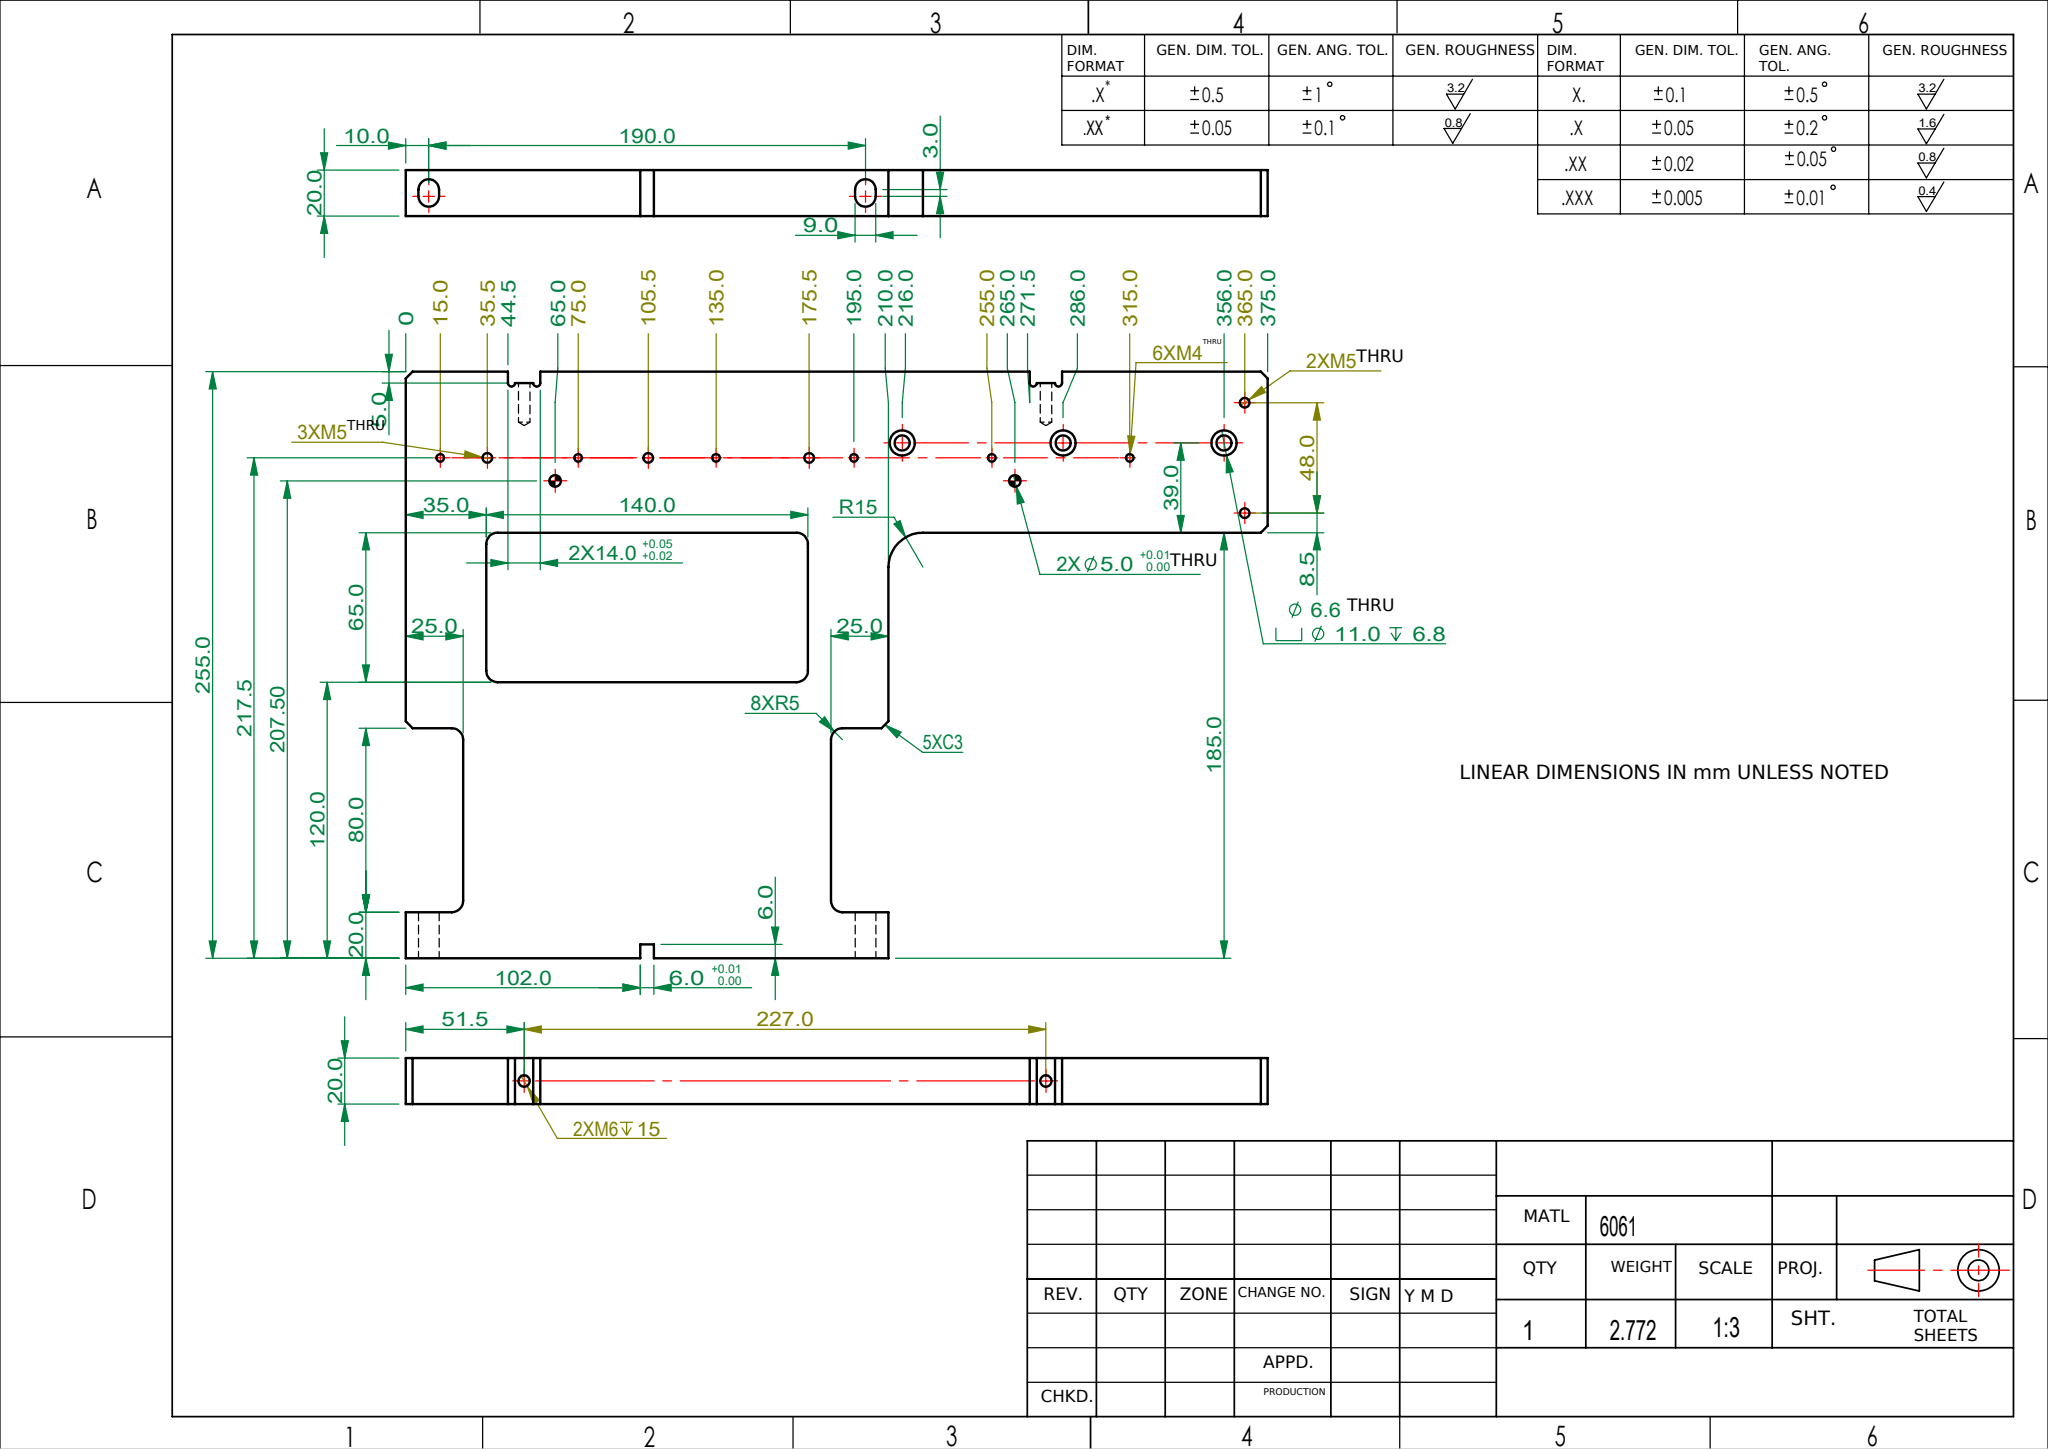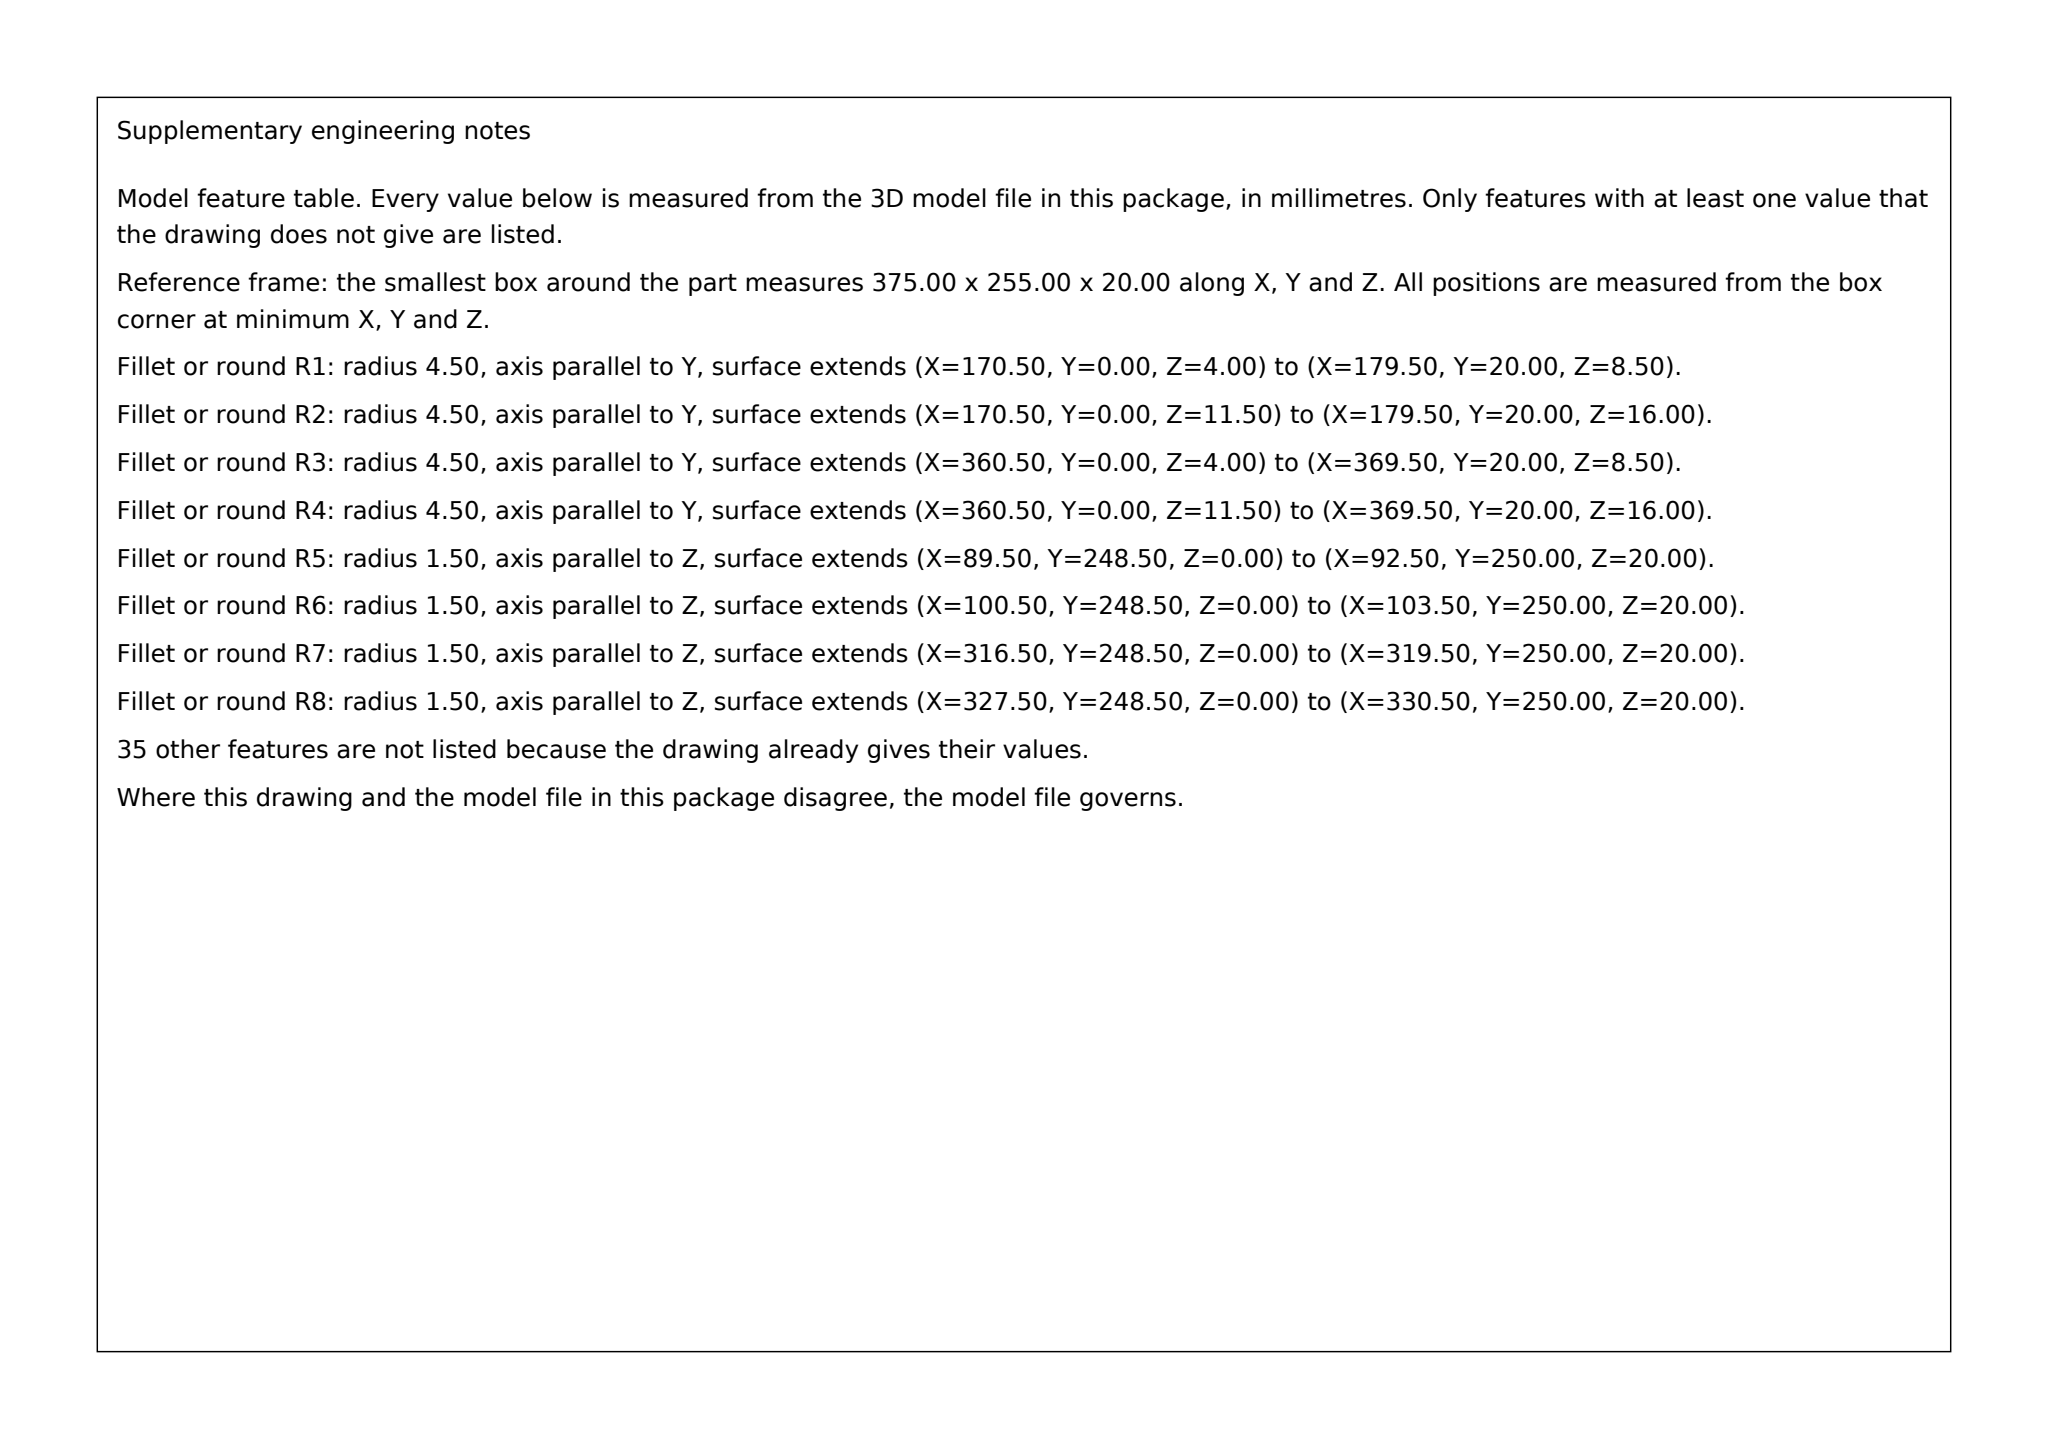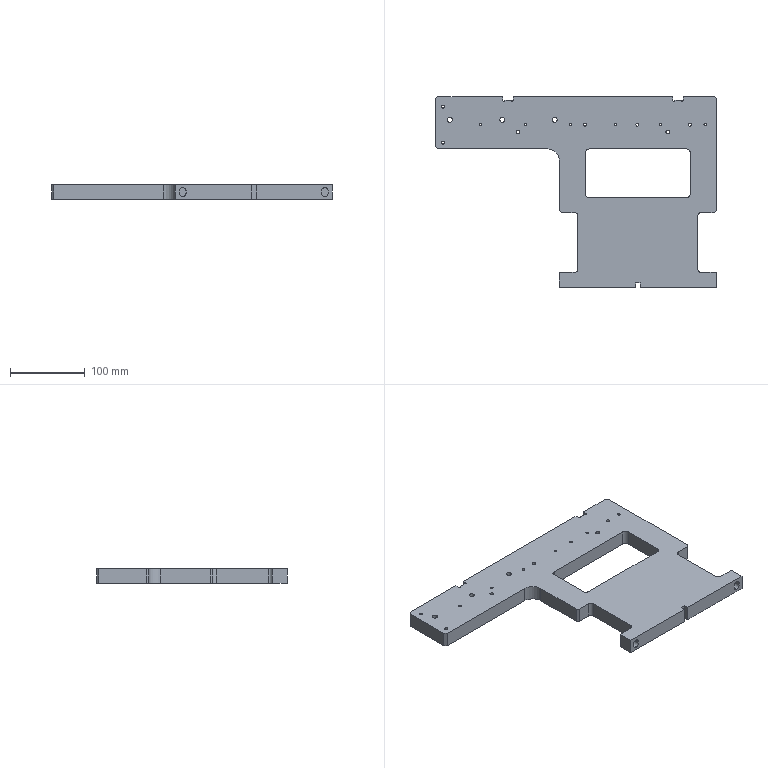Part | SolidWorks | mm | material 6061 | 1 solid | 109 faces | box 375 x 255 x 20 mm | volume 1026769 mm3 | cylinder 61 | plane 44 | cone 4 | commonest cylinder face diameters 3.3 x12 4.2 x10 5 x8 10 x8 11 x6 6.6 x6 9 x6 3 x4
build123d program:
from build123d import *

# Parameters (mm, degrees)
SKETCH1_W                                          = 375
SKETCH1_H                                          = 255
BOSS_EXTRUDE1_DEPTH                                = 20
M5_TAPPED_HOLE1_D                                  = 4.2
M4_TAPPED_HOLE1_D                                  = 3.3
LPATTERN1_COUNT                                    = 6
LPATTERN1_PITCH                                    = 60
SKETCH6_W                                          = 165
SKETCH6_H                                          = 185
CUT_EXTRUDE1_DEPTH                                 = 70
SKETCH7_W                                          = 25
SKETCH7_H                                          = 80
CUT_EXTRUDE2_DEPTH                                 = 70
F_8_5_8_5_DIAMETER_HOLE1_REACH                     = 447.365
F_8_5_8_5_DIAMETER_HOLE1_BORE_R                    = 4.25
CUT_EXTRUDE3_DEPTH                                 = 70
HOLE_SIZE_ACCORDING_TO_TYPE_1_OF_HEXAG_D           = 6.6
HOLE_SIZE_ACCORDING_TO_TYPE_1_OF_HEXAG_CBORE_D     = 11
HOLE_SIZE_ACCORDING_TO_TYPE_1_OF_HEXAG_CBORE_DEPTH = 6.8
LPATTERN2_COUNT                                    = 3
LPATTERN2_PITCH                                    = 70
SKETCH14_W                                         = 140
SKETCH14_H                                         = 65
CUT_EXTRUDE4_DEPTH                                 = 79
FILLET1_R                                          = 5
SKETCH17_W                                         = 14
SKETCH17_H                                         = 10
CUT_EXTRUDE5_DEPTH                                 = 37
LPATTERN3_COUNT                                    = 2
LPATTERN3_PITCH                                    = 227
SKETCH20_W                                         = 6
SKETCH20_H                                         = 12
CUT_EXTRUDE6_DEPTH                                 = 37
SIZE_MM_DOWEL_PIN_HOLE_1_D                         = 5
FILLET2_R                                          = 15
CHAMFER1_SIZE                                      = 3
FILLET3_R                                          = 5
M5_TAPPED_HOLE2_D                                  = 4.2
LPATTERN4_COUNT                                    = 3
LPATTERN4_PITCH                                    = 70
SKETCH25_R                                         = 1.5
CUT_EXTRUDE7_DEPTH                                 = 36


with BuildPart() as part:
    # Sketch1 → Boss-Extrude1 (new body)
    with BuildSketch(Plane.XY):
        Rectangle(SKETCH1_W, SKETCH1_H)
    extrude(amount=BOSS_EXTRUDE1_DEPTH)

    # M5 Tapped Hole1 (through all)
    with Locations(Plane(origin=(-177.5, 114, 20), x_dir=(1, 0, 0), z_dir=(0, 0, 1))):
        with Locations((0, 0), (0, -48)):
            Hole(M5_TAPPED_HOLE1_D / 2)

    # M4 Tapped Hole1 (through all)
    with Locations(Plane(origin=(-127.5, 90, 20), x_dir=(1, 0, 0), z_dir=(0, 0, 1))):
        with Locations((0, 0)):
            m4_tapped_hole1 = Hole(M4_TAPPED_HOLE1_D / 2)

    # LPattern1: M4 Tapped Hole1 ×6
    with Locations(*[(i * LPATTERN1_PITCH, 0, 0) for i in range(1, LPATTERN1_COUNT)]):
        add(m4_tapped_hole1, mode=Mode.SUBTRACT)

    # Sketch6 → Cut-Extrude1 (cut)
    with BuildSketch(Plane.XY.offset(20)):
        with Locations((-105, -35)):
            Rectangle(SKETCH6_W, SKETCH6_H)
    extrude(amount=-CUT_EXTRUDE1_DEPTH, mode=Mode.SUBTRACT)

    # Sketch7 → Cut-Extrude2 (cut)
    with BuildSketch(Plane.XY.offset(20)):
        with Locations((-10, -67.5)):
            Rectangle(SKETCH7_W, SKETCH7_H)
        with Locations((175, -67.5)):
            Rectangle(SKETCH7_W, SKETCH7_H)
    extrude(amount=-CUT_EXTRUDE2_DEPTH, mode=Mode.SUBTRACT)

    # 8.5 _8.5_ Diameter Hole1 bore (on position points) → 8.5 _8.5_ Diameter Hole1 (cut, up to next)
    with BuildSketch(Plane(origin=(177.5, -127.5, 10), x_dir=(0, 0, -1), z_dir=(0, -1, 0)), mode=Mode.PRIVATE) as f_8_5_8_5_diameter_hole1_sk1:
        Circle(F_8_5_8_5_DIAMETER_HOLE1_BORE_R)
    f_8_5_8_5_diameter_hole1_tool1 = extrude(f_8_5_8_5_diameter_hole1_sk1.sketch, amount=-F_8_5_8_5_DIAMETER_HOLE1_REACH, mode=Mode.PRIVATE) & part.part
    # 8.5 _8.5_ Diameter Hole1 bore (on position points) → 8.5 _8.5_ Diameter Hole1 (cut, up to next)
    with BuildSketch(Plane(origin=(177.5, -127.5, 10), x_dir=(0, 0, -1), z_dir=(0, -1, 0)), mode=Mode.PRIVATE) as f_8_5_8_5_diameter_hole1_sk2:
        with Locations((0, -190)):
            Circle(F_8_5_8_5_DIAMETER_HOLE1_BORE_R)
    f_8_5_8_5_diameter_hole1_tool2 = extrude(f_8_5_8_5_diameter_hole1_sk2.sketch, amount=-F_8_5_8_5_DIAMETER_HOLE1_REACH, mode=Mode.PRIVATE) & part.part
    add(f_8_5_8_5_diameter_hole1_tool1.solids().sort_by_distance((177.5, -127.5, 10))[0], mode=Mode.SUBTRACT)
    add(f_8_5_8_5_diameter_hole1_tool2.solids().sort_by_distance((-12.5, -127.5, 10))[0], mode=Mode.SUBTRACT)

    # Sketch11 → Cut-Extrude3 (cut)
    with BuildSketch(Plane.XZ.offset(127.5)):
        with BuildLine():
            Line((-17, 8.5), (-17, 11.5))
            ThreePointArc((-17, 11.5), (-12.5, 16), (-8, 11.5))
            Line((-8, 11.5), (-8, 8.5))
            ThreePointArc((-8, 8.5), (-12.5, 4), (-17, 8.5))
        make_face()
        with BuildLine():
            Line((173, 8.5), (173, 11.5))
            ThreePointArc((173, 11.5), (177.5, 16), (182, 11.5))
            Line((182, 11.5), (182, 8.5))
            ThreePointArc((182, 8.5), (177.5, 4), (173, 8.5))
        make_face()
    extrude(amount=-CUT_EXTRUDE3_DEPTH, mode=Mode.SUBTRACT)

    # Hole Size _according to_ Type 1 of Hexag (through all)
    with Locations(Plane(origin=(-28.5, 96.5, 0), x_dir=(-1, 0, 0), z_dir=(0, 0, -1))):
        with Locations((0, 0)):
            hole_size_according_to_type_1_of_hexag = CounterBoreHole(HOLE_SIZE_ACCORDING_TO_TYPE_1_OF_HEXAG_D / 2, HOLE_SIZE_ACCORDING_TO_TYPE_1_OF_HEXAG_CBORE_D / 2, HOLE_SIZE_ACCORDING_TO_TYPE_1_OF_HEXAG_CBORE_DEPTH)

    # LPattern2: Hole Size _according to_ Type 1 of Hexag ×3
    with Locations(*[(-i * LPATTERN2_PITCH, 0, 0) for i in range(1, LPATTERN2_COUNT)]):
        add(hole_size_according_to_type_1_of_hexag, mode=Mode.SUBTRACT)

    # Sketch14 → Cut-Extrude4 (cut)
    with BuildSketch(Plane.XY.offset(20)):
        with Locations((82.5, 25)):
            Rectangle(SKETCH14_W, SKETCH14_H)
    extrude(amount=-CUT_EXTRUDE4_DEPTH, mode=Mode.SUBTRACT)

    # Fillet1
    fillet1_edges = [part.edges().sort_by_distance(p)[0] for p in [
        (152.5, 57.5, 10),
        (152.5, -7.5, 10),
        (12.5, -7.5, 10),
        (12.5, 57.5, 10),
    ]]
    fillet(fillet1_edges, radius=FILLET1_R)

    # Sketch17 → Cut-Extrude5 (cut)
    with BuildSketch(Plane.XY.offset(20)):
        with Locations((136, 127.5)):
            Rectangle(SKETCH17_W, SKETCH17_H)
    cut_extrude5 = extrude(amount=-CUT_EXTRUDE5_DEPTH, mode=Mode.SUBTRACT)

    # Sketch19 → M6 Tapped Hole1 (revolve, cut)
    with BuildSketch(Plane(origin=(136, 122.5, 10), x_dir=(0, 0, 1), z_dir=(1, 0, 0))):
        Polygon((0, 0), (0, 18.502), (2.5, 17), (2.5, 0), align=None)
    m6_tapped_hole1 = revolve(axis=Axis((136, 128.85, 10), (0, -1, 0)), mode=Mode.SUBTRACT)

    # LPattern3: Cut-Extrude5, M6 Tapped Hole1 ×2
    with Locations(*[(-i * LPATTERN3_PITCH, 0, 0) for i in range(1, LPATTERN3_COUNT)]):
        add(cut_extrude5, mode=Mode.SUBTRACT)
        add(m6_tapped_hole1, mode=Mode.SUBTRACT)

    # Sketch20 → Cut-Extrude6 (cut)
    with BuildSketch(Plane.XY.offset(20)):
        with Locations((82.5, -127.5)):
            Rectangle(SKETCH20_W, SKETCH20_H)
    extrude(amount=-CUT_EXTRUDE6_DEPTH, mode=Mode.SUBTRACT)

    # Size mm Dowel Pin Hole 1 (through all)
    with Locations(Plane(origin=(-77.5, 80, 20), x_dir=(1, 0, 0), z_dir=(0, 0, 1))):
        with Locations((0, 0), (200, 0)):
            Hole(SIZE_MM_DOWEL_PIN_HOLE_1_D / 2)

    # Fillet2
    fillet2_edges = [part.edges().sort_by_distance(p)[0] for p in [
        (-22.5, 57.5, 10),
    ]]
    fillet(fillet2_edges, radius=FILLET2_R)

    # Chamfer1
    chamfer1_edges = [part.edges().sort_by_distance(p)[0] for p in [
        (-187.5, 57.5, 10),
        (-22.5, -27.5, 10),
        (-187.5, 127.5, 10),
        (187.5, 127.5, 10),
        (187.5, -27.5, 10),
    ]]
    chamfer(chamfer1_edges, length=CHAMFER1_SIZE)

    # Fillet3
    fillet3_edges = [part.edges().sort_by_distance(p)[0] for p in [
        (2.5, -27.5, 10),
        (2.5, -107.5, 10),
        (162.5, -107.5, 10),
        (162.5, -27.5, 10),
    ]]
    fillet(fillet3_edges, radius=FILLET3_R)

    # M5 Tapped Hole2 (through all)
    with Locations(Plane(origin=(152, 90, 20), x_dir=(1, 0, 0), z_dir=(0, 0, 1))):
        with Locations((0, 0)):
            m5_tapped_hole2 = Hole(M5_TAPPED_HOLE2_D / 2)

    # LPattern4: M5 Tapped Hole2 ×3
    with Locations(*[(-i * LPATTERN4_PITCH, 0, 0) for i in range(1, LPATTERN4_COUNT)]):
        add(m5_tapped_hole2, mode=Mode.SUBTRACT)

    # Sketch25 → Cut-Extrude7 (cut)
    with BuildSketch(Plane(origin=(0, 0, 0), x_dir=(-1, 0, 0), z_dir=(0, 0, -1))):
        with Locations((-141.5, 122.5)):
            Circle(SKETCH25_R)
        with Locations((-130.5, 122.5)):
            Circle(SKETCH25_R)
        with Locations((85.5, 122.5)):
            Circle(SKETCH25_R)
        with Locations((96.5, 122.5)):
            Circle(SKETCH25_R)
    extrude(amount=-CUT_EXTRUDE7_DEPTH, mode=Mode.SUBTRACT)


solid = part.part